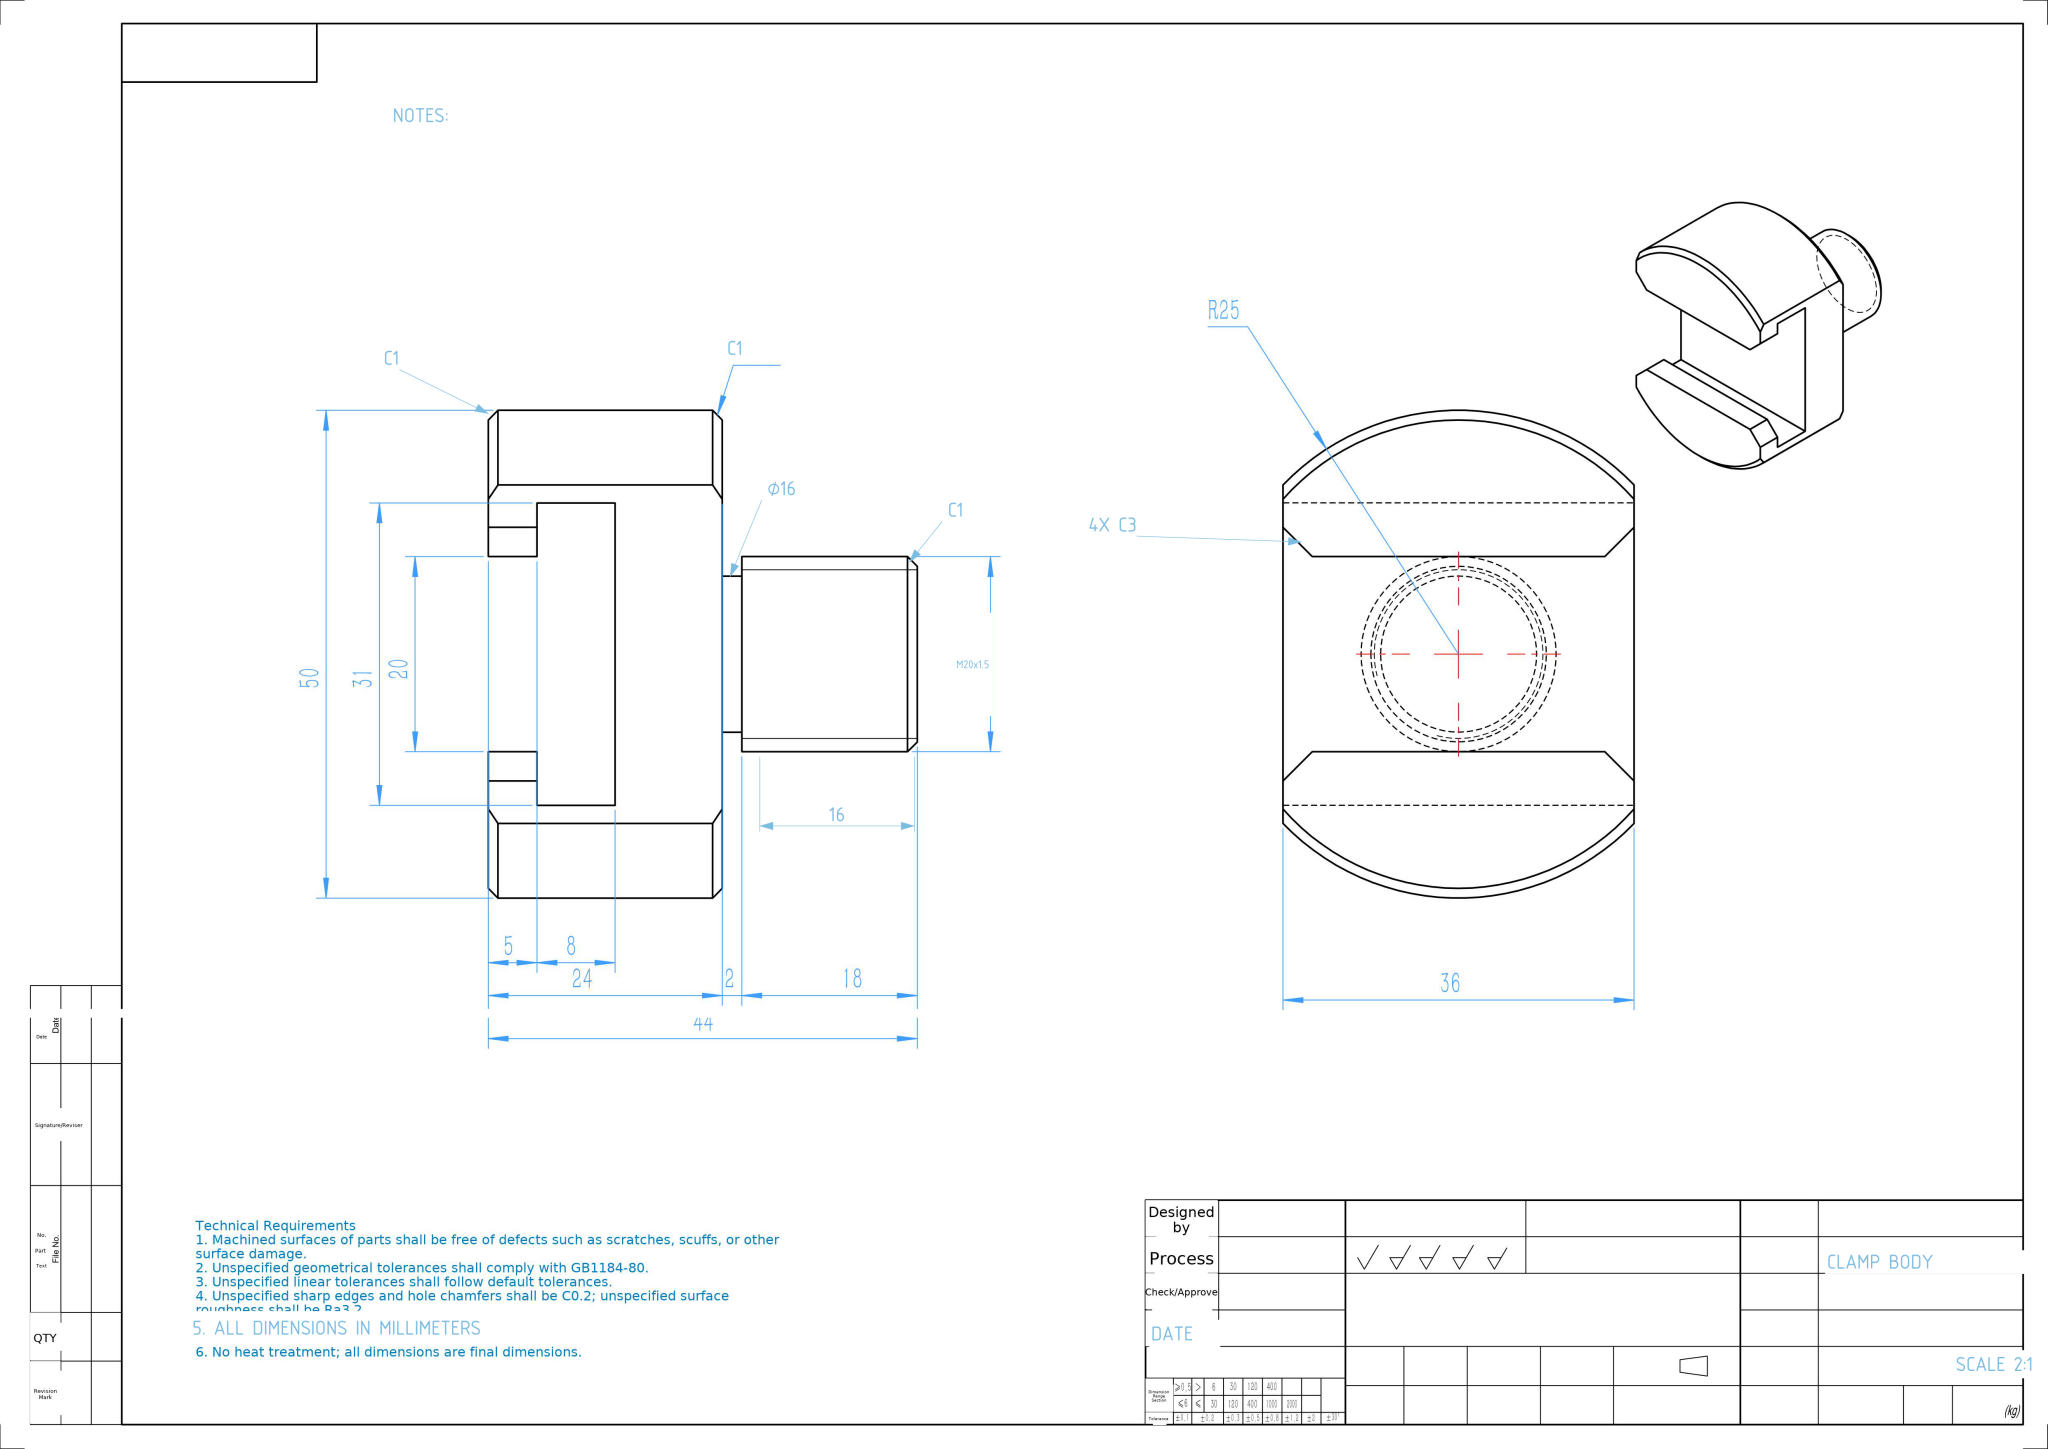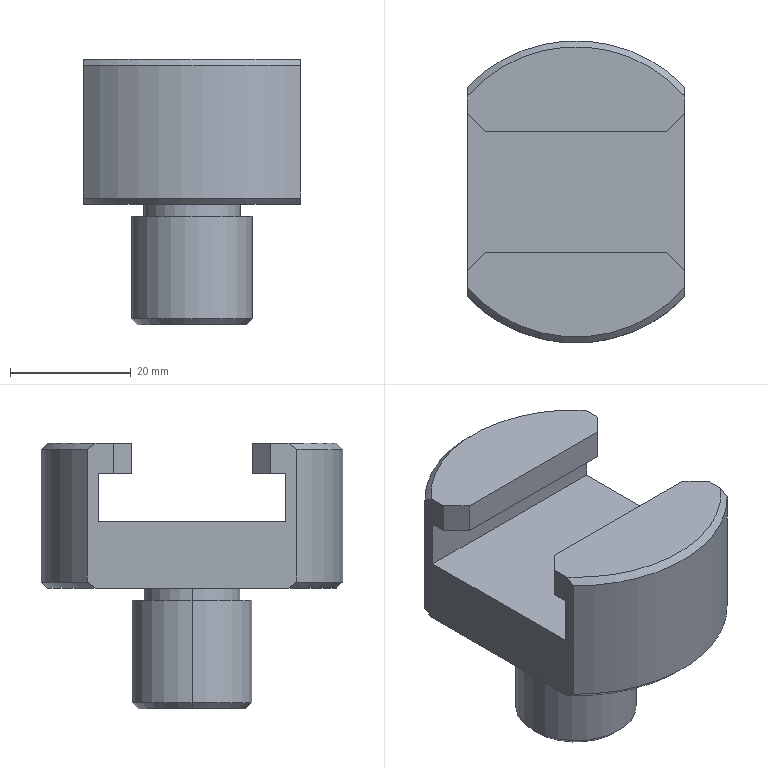Part | NX | mm | 1 solid | 30 faces | box 36 x 50 x 44 mm | volume 32432 mm3 | plane 18 | cylinder 6 | cone 6 | commonest cylinder face diameters 20 x2 16 x2 50 x2
STEP:
#1=CARTESIAN_POINT('',(10.,0.,-19.));
#2=VERTEX_POINT('',#1);
#3=CARTESIAN_POINT('',(-10.,0.,-19.));
#4=VERTEX_POINT('',#3);
#5=CARTESIAN_POINT('',(0.,0.,-19.));
#6=DIRECTION('',(0.,0.,1.));
#7=DIRECTION('',(-1.,0.,0.));
#8=AXIS2_PLACEMENT_3D('',#5,#6,#7);
#9=CIRCLE('',#8,10.);
#10=EDGE_CURVE('',#2,#4,#9,.T.);
#11=ORIENTED_EDGE('',*,*,#10,.T.);
#12=CARTESIAN_POINT('',(-10.,0.,-2.));
#13=VERTEX_POINT('',#12);
#14=CARTESIAN_POINT('',(-10.,0.,-20.));
#15=DIRECTION('',(0.,0.,1.));
#16=VECTOR('',#15,1000.);
#17=LINE('',#14,#16);
#18=EDGE_CURVE('',#4,#13,#17,.T.);
#19=ORIENTED_EDGE('',*,*,#18,.T.);
#20=CARTESIAN_POINT('',(10.,0.,-2.));
#21=VERTEX_POINT('',#20);
#22=CARTESIAN_POINT('',(0.,0.,-2.));
#23=DIRECTION('',(0.,0.,-1.));
#24=DIRECTION('',(-1.,0.,0.));
#25=AXIS2_PLACEMENT_3D('',#22,#23,#24);
#26=CIRCLE('',#25,10.);
#27=EDGE_CURVE('',#13,#21,#26,.T.);
#28=ORIENTED_EDGE('',*,*,#27,.T.);
#29=CARTESIAN_POINT('',(10.,0.,-20.));
#30=DIRECTION('',(0.,0.,1.));
#31=VECTOR('',#30,1000.);
#32=LINE('',#29,#31);
#33=EDGE_CURVE('',#2,#21,#32,.T.);
#34=ORIENTED_EDGE('',*,*,#33,.F.);
#35=EDGE_LOOP('',(#11,#19,#28,#34));
#36=FACE_OUTER_BOUND('',#35,.T.);
#37=CARTESIAN_POINT('',(0.,0.,-20.));
#38=DIRECTION('',(0.,0.,1.));
#39=DIRECTION('',(1.,0.,0.));
#40=AXIS2_PLACEMENT_3D('',#37,#38,#39);
#41=CYLINDRICAL_SURFACE('',#40,10.);
#42=ADVANCED_FACE('',(#36),#41,.T.);
#43=CARTESIAN_POINT('',(-9.,0.,-20.));
#44=VERTEX_POINT('',#43);
#45=CARTESIAN_POINT('',(9.,0.,-20.));
#46=VERTEX_POINT('',#45);
#47=CARTESIAN_POINT('',(0.,0.,-20.));
#48=DIRECTION('',(0.,0.,-1.));
#49=DIRECTION('',(-1.,0.,0.));
#50=AXIS2_PLACEMENT_3D('',#47,#48,#49);
#51=CIRCLE('',#50,9.);
#52=EDGE_CURVE('',#44,#46,#51,.T.);
#53=ORIENTED_EDGE('',*,*,#52,.F.);
#54=CARTESIAN_POINT('',(-9.,0.,-20.));
#55=DIRECTION('',(-0.7071,0.,0.7071));
#56=VECTOR('',#55,1000.);
#57=LINE('',#54,#56);
#58=EDGE_CURVE('',#44,#4,#57,.T.);
#59=ORIENTED_EDGE('',*,*,#58,.T.);
#60=ORIENTED_EDGE('',*,*,#10,.F.);
#61=CARTESIAN_POINT('',(9.,0.,-20.));
#62=DIRECTION('',(0.7071,0.,0.7071));
#63=VECTOR('',#62,1000.);
#64=LINE('',#61,#63);
#65=EDGE_CURVE('',#46,#2,#64,.T.);
#66=ORIENTED_EDGE('',*,*,#65,.F.);
#67=EDGE_LOOP('',(#53,#59,#60,#66));
#68=FACE_OUTER_BOUND('',#67,.T.);
#69=CARTESIAN_POINT('',(0.,0.,-20.));
#70=DIRECTION('',(0.,0.,1.));
#71=DIRECTION('',(1.,0.,0.));
#72=AXIS2_PLACEMENT_3D('',#69,#70,#71);
#73=CONICAL_SURFACE('',#72,9.,0.7854);
#74=ADVANCED_FACE('',(#68),#73,.T.);
#75=CARTESIAN_POINT('',(-8.,0.,0.));
#76=VERTEX_POINT('',#75);
#77=CARTESIAN_POINT('',(8.,0.,0.));
#78=VERTEX_POINT('',#77);
#79=CARTESIAN_POINT('',(0.,0.,0.));
#80=DIRECTION('',(0.,0.,-1.));
#81=DIRECTION('',(-1.,0.,0.));
#82=AXIS2_PLACEMENT_3D('',#79,#80,#81);
#83=CIRCLE('',#82,8.);
#84=EDGE_CURVE('',#76,#78,#83,.T.);
#85=ORIENTED_EDGE('',*,*,#84,.T.);
#86=CARTESIAN_POINT('',(8.,0.,-2.));
#87=VERTEX_POINT('',#86);
#88=CARTESIAN_POINT('',(8.,0.,-19.));
#89=DIRECTION('',(0.,0.,-1.));
#90=VECTOR('',#89,1000.);
#91=LINE('',#88,#90);
#92=EDGE_CURVE('',#78,#87,#91,.T.);
#93=ORIENTED_EDGE('',*,*,#92,.T.);
#94=CARTESIAN_POINT('',(-8.,0.,-2.));
#95=VERTEX_POINT('',#94);
#96=CARTESIAN_POINT('',(0.,0.,-2.));
#97=DIRECTION('',(0.,0.,-1.));
#98=DIRECTION('',(-1.,0.,0.));
#99=AXIS2_PLACEMENT_3D('',#96,#97,#98);
#100=CIRCLE('',#99,8.);
#101=EDGE_CURVE('',#95,#87,#100,.T.);
#102=ORIENTED_EDGE('',*,*,#101,.F.);
#103=CARTESIAN_POINT('',(-8.,0.,-19.));
#104=DIRECTION('',(0.,0.,-1.));
#105=VECTOR('',#104,1000.);
#106=LINE('',#103,#105);
#107=EDGE_CURVE('',#76,#95,#106,.T.);
#108=ORIENTED_EDGE('',*,*,#107,.F.);
#109=EDGE_LOOP('',(#85,#93,#102,#108));
#110=FACE_OUTER_BOUND('',#109,.T.);
#111=CARTESIAN_POINT('',(0.,0.,-19.));
#112=DIRECTION('',(0.,0.,-1.));
#113=DIRECTION('',(-1.,0.,0.));
#114=AXIS2_PLACEMENT_3D('',#111,#112,#113);
#115=CYLINDRICAL_SURFACE('',#114,8.);
#116=ADVANCED_FACE('',(#110),#115,.T.);
#117=CARTESIAN_POINT('',(18.,-17.349,1.));
#118=VERTEX_POINT('',#117);
#119=CARTESIAN_POINT('',(18.,-17.349,23.));
#120=VERTEX_POINT('',#119);
#121=CARTESIAN_POINT('',(18.,-17.349,24.));
#122=DIRECTION('',(0.,0.,1.));
#123=VECTOR('',#122,1000.);
#124=LINE('',#121,#123);
#125=EDGE_CURVE('',#118,#120,#124,.T.);
#126=ORIENTED_EDGE('',*,*,#125,.T.);
#127=CARTESIAN_POINT('',(-18.,-17.349,23.));
#128=VERTEX_POINT('',#127);
#129=CARTESIAN_POINT('',(0.,0.,23.));
#130=DIRECTION('',(0.,0.,-1.));
#131=DIRECTION('',(1.,0.,0.));
#132=AXIS2_PLACEMENT_3D('',#129,#130,#131);
#133=CIRCLE('',#132,25.);
#134=EDGE_CURVE('',#120,#128,#133,.T.);
#135=ORIENTED_EDGE('',*,*,#134,.T.);
#136=CARTESIAN_POINT('',(-18.,-17.349,1.));
#137=VERTEX_POINT('',#136);
#138=CARTESIAN_POINT('',(-18.,-17.349,24.));
#139=DIRECTION('',(0.,0.,-1.));
#140=VECTOR('',#139,1000.);
#141=LINE('',#138,#140);
#142=EDGE_CURVE('',#128,#137,#141,.T.);
#143=ORIENTED_EDGE('',*,*,#142,.T.);
#144=CARTESIAN_POINT('',(0.,0.,1.));
#145=DIRECTION('',(0.,0.,1.));
#146=DIRECTION('',(1.,0.,0.));
#147=AXIS2_PLACEMENT_3D('',#144,#145,#146);
#148=CIRCLE('',#147,25.);
#149=EDGE_CURVE('',#137,#118,#148,.T.);
#150=ORIENTED_EDGE('',*,*,#149,.T.);
#151=EDGE_LOOP('',(#126,#135,#143,#150));
#152=FACE_OUTER_BOUND('',#151,.T.);
#153=CARTESIAN_POINT('',(0.,0.,24.));
#154=DIRECTION('',(0.,0.,-1.));
#155=DIRECTION('',(-1.,0.,0.));
#156=AXIS2_PLACEMENT_3D('',#153,#154,#155);
#157=CYLINDRICAL_SURFACE('',#156,25.);
#158=ADVANCED_FACE('',(#152),#157,.T.);
#159=CARTESIAN_POINT('',(-18.,13.,24.));
#160=VERTEX_POINT('',#159);
#161=CARTESIAN_POINT('',(-18.,15.875,24.));
#162=VERTEX_POINT('',#161);
#163=CARTESIAN_POINT('',(-18.,25.313,24.));
#164=DIRECTION('',(0.,1.,0.));
#165=VECTOR('',#164,1000.);
#166=LINE('',#163,#165);
#167=EDGE_CURVE('',#160,#162,#166,.T.);
#168=ORIENTED_EDGE('',*,*,#167,.F.);
#169=CARTESIAN_POINT('',(-15.,10.,24.));
#170=VERTEX_POINT('',#169);
#171=CARTESIAN_POINT('',(-2.5,-2.5,24.));
#172=DIRECTION('',(0.7071,-0.7071,0.));
#173=VECTOR('',#172,1000.);
#174=LINE('',#171,#173);
#175=EDGE_CURVE('',#160,#170,#174,.T.);
#176=ORIENTED_EDGE('',*,*,#175,.T.);
#177=CARTESIAN_POINT('',(15.,10.,24.));
#178=VERTEX_POINT('',#177);
#179=CARTESIAN_POINT('',(0.,10.,24.));
#180=DIRECTION('',(-1.,0.,0.));
#181=VECTOR('',#180,1000.);
#182=LINE('',#179,#181);
#183=EDGE_CURVE('',#178,#170,#182,.T.);
#184=ORIENTED_EDGE('',*,*,#183,.F.);
#185=CARTESIAN_POINT('',(18.,13.,24.));
#186=VERTEX_POINT('',#185);
#187=CARTESIAN_POINT('',(2.5,-2.5,24.));
#188=DIRECTION('',(0.7071,0.7071,0.));
#189=VECTOR('',#188,1000.);
#190=LINE('',#187,#189);
#191=EDGE_CURVE('',#178,#186,#190,.T.);
#192=ORIENTED_EDGE('',*,*,#191,.T.);
#193=CARTESIAN_POINT('',(18.,15.875,24.));
#194=VERTEX_POINT('',#193);
#195=CARTESIAN_POINT('',(18.,25.314,24.));
#196=DIRECTION('',(0.,-1.,0.));
#197=VECTOR('',#196,1000.);
#198=LINE('',#195,#197);
#199=EDGE_CURVE('',#194,#186,#198,.T.);
#200=ORIENTED_EDGE('',*,*,#199,.F.);
#201=CARTESIAN_POINT('',(0.,0.,24.));
#202=DIRECTION('',(0.,0.,1.));
#203=DIRECTION('',(1.,0.,0.));
#204=AXIS2_PLACEMENT_3D('',#201,#202,#203);
#205=CIRCLE('',#204,24.);
#206=EDGE_CURVE('',#194,#162,#205,.T.);
#207=ORIENTED_EDGE('',*,*,#206,.T.);
#208=EDGE_LOOP('',(#168,#176,#184,#192,#200,#207));
#209=FACE_OUTER_BOUND('',#208,.T.);
#210=CARTESIAN_POINT('',(0.,0.,24.));
#211=DIRECTION('',(0.,0.,1.));
#212=DIRECTION('',(1.,0.,0.));
#213=AXIS2_PLACEMENT_3D('',#210,#211,#212);
#214=PLANE('',#213);
#215=ADVANCED_FACE('',(#209),#214,.T.);
#216=CARTESIAN_POINT('',(-18.,17.349,1.));
#217=VERTEX_POINT('',#216);
#218=CARTESIAN_POINT('',(-18.,17.349,23.));
#219=VERTEX_POINT('',#218);
#220=CARTESIAN_POINT('',(-18.,17.349,24.));
#221=DIRECTION('',(0.,0.,1.));
#222=VECTOR('',#221,1000.);
#223=LINE('',#220,#222);
#224=EDGE_CURVE('',#217,#219,#223,.T.);
#225=ORIENTED_EDGE('',*,*,#224,.T.);
#226=CARTESIAN_POINT('',(18.,17.349,23.));
#227=VERTEX_POINT('',#226);
#228=CARTESIAN_POINT('',(0.,0.,23.));
#229=DIRECTION('',(0.,0.,-1.));
#230=DIRECTION('',(1.,0.,0.));
#231=AXIS2_PLACEMENT_3D('',#228,#229,#230);
#232=CIRCLE('',#231,25.);
#233=EDGE_CURVE('',#219,#227,#232,.T.);
#234=ORIENTED_EDGE('',*,*,#233,.T.);
#235=CARTESIAN_POINT('',(18.,17.349,1.));
#236=VERTEX_POINT('',#235);
#237=CARTESIAN_POINT('',(18.,17.349,24.));
#238=DIRECTION('',(0.,0.,-1.));
#239=VECTOR('',#238,1000.);
#240=LINE('',#237,#239);
#241=EDGE_CURVE('',#227,#236,#240,.T.);
#242=ORIENTED_EDGE('',*,*,#241,.T.);
#243=CARTESIAN_POINT('',(0.,0.,1.));
#244=DIRECTION('',(0.,0.,1.));
#245=DIRECTION('',(1.,0.,0.));
#246=AXIS2_PLACEMENT_3D('',#243,#244,#245);
#247=CIRCLE('',#246,25.);
#248=EDGE_CURVE('',#236,#217,#247,.T.);
#249=ORIENTED_EDGE('',*,*,#248,.T.);
#250=EDGE_LOOP('',(#225,#234,#242,#249));
#251=FACE_OUTER_BOUND('',#250,.T.);
#252=CARTESIAN_POINT('',(0.,0.,24.));
#253=DIRECTION('',(0.,0.,-1.));
#254=DIRECTION('',(-1.,0.,0.));
#255=AXIS2_PLACEMENT_3D('',#252,#253,#254);
#256=CYLINDRICAL_SURFACE('',#255,25.);
#257=ADVANCED_FACE('',(#251),#256,.T.);
#258=CARTESIAN_POINT('',(-15.,-10.,24.));
#259=VERTEX_POINT('',#258);
#260=CARTESIAN_POINT('',(15.,-10.,24.));
#261=VERTEX_POINT('',#260);
#262=CARTESIAN_POINT('',(0.,-10.,24.));
#263=DIRECTION('',(1.,0.,0.));
#264=VECTOR('',#263,1000.);
#265=LINE('',#262,#264);
#266=EDGE_CURVE('',#259,#261,#265,.T.);
#267=ORIENTED_EDGE('',*,*,#266,.F.);
#268=CARTESIAN_POINT('',(-18.,-13.,24.));
#269=VERTEX_POINT('',#268);
#270=CARTESIAN_POINT('',(-2.5,2.5,24.));
#271=DIRECTION('',(-0.7071,-0.7071,0.));
#272=VECTOR('',#271,1000.);
#273=LINE('',#270,#272);
#274=EDGE_CURVE('',#259,#269,#273,.T.);
#275=ORIENTED_EDGE('',*,*,#274,.T.);
#276=CARTESIAN_POINT('',(-18.,-15.875,24.));
#277=VERTEX_POINT('',#276);
#278=CARTESIAN_POINT('',(-18.,25.313,24.));
#279=DIRECTION('',(0.,1.,0.));
#280=VECTOR('',#279,1000.);
#281=LINE('',#278,#280);
#282=EDGE_CURVE('',#277,#269,#281,.T.);
#283=ORIENTED_EDGE('',*,*,#282,.F.);
#284=CARTESIAN_POINT('',(18.,-15.875,24.));
#285=VERTEX_POINT('',#284);
#286=CARTESIAN_POINT('',(0.,0.,24.));
#287=DIRECTION('',(0.,0.,1.));
#288=DIRECTION('',(1.,0.,0.));
#289=AXIS2_PLACEMENT_3D('',#286,#287,#288);
#290=CIRCLE('',#289,24.);
#291=EDGE_CURVE('',#277,#285,#290,.T.);
#292=ORIENTED_EDGE('',*,*,#291,.T.);
#293=CARTESIAN_POINT('',(18.,-13.,24.));
#294=VERTEX_POINT('',#293);
#295=CARTESIAN_POINT('',(18.,25.314,24.));
#296=DIRECTION('',(0.,-1.,0.));
#297=VECTOR('',#296,1000.);
#298=LINE('',#295,#297);
#299=EDGE_CURVE('',#294,#285,#298,.T.);
#300=ORIENTED_EDGE('',*,*,#299,.F.);
#301=CARTESIAN_POINT('',(2.5,2.5,24.));
#302=DIRECTION('',(-0.7071,0.7071,0.));
#303=VECTOR('',#302,1000.);
#304=LINE('',#301,#303);
#305=EDGE_CURVE('',#294,#261,#304,.T.);
#306=ORIENTED_EDGE('',*,*,#305,.T.);
#307=EDGE_LOOP('',(#267,#275,#283,#292,#300,#306));
#308=FACE_OUTER_BOUND('',#307,.T.);
#309=CARTESIAN_POINT('',(0.,0.,24.));
#310=DIRECTION('',(0.,0.,1.));
#311=DIRECTION('',(1.,0.,0.));
#312=AXIS2_PLACEMENT_3D('',#309,#310,#311);
#313=PLANE('',#312);
#314=ADVANCED_FACE('',(#308),#313,.T.);
#315=CARTESIAN_POINT('',(18.,15.875,0.));
#316=VERTEX_POINT('',#315);
#317=CARTESIAN_POINT('',(18.,-15.875,0.));
#318=VERTEX_POINT('',#317);
#319=CARTESIAN_POINT('',(18.,0.,0.));
#320=DIRECTION('',(0.,-1.,0.));
#321=VECTOR('',#320,1000.);
#322=LINE('',#319,#321);
#323=EDGE_CURVE('',#316,#318,#322,.T.);
#324=ORIENTED_EDGE('',*,*,#323,.T.);
#325=CARTESIAN_POINT('',(-18.,-15.875,0.));
#326=VERTEX_POINT('',#325);
#327=CARTESIAN_POINT('',(0.,0.,0.));
#328=DIRECTION('',(0.,0.,-1.));
#329=DIRECTION('',(1.,0.,0.));
#330=AXIS2_PLACEMENT_3D('',#327,#328,#329);
#331=CIRCLE('',#330,24.);
#332=EDGE_CURVE('',#318,#326,#331,.T.);
#333=ORIENTED_EDGE('',*,*,#332,.T.);
#334=CARTESIAN_POINT('',(-18.,15.875,0.));
#335=VERTEX_POINT('',#334);
#336=CARTESIAN_POINT('',(-18.,0.,0.));
#337=DIRECTION('',(0.,1.,0.));
#338=VECTOR('',#337,1000.);
#339=LINE('',#336,#338);
#340=EDGE_CURVE('',#326,#335,#339,.T.);
#341=ORIENTED_EDGE('',*,*,#340,.T.);
#342=CARTESIAN_POINT('',(0.,0.,0.));
#343=DIRECTION('',(0.,0.,-1.));
#344=DIRECTION('',(1.,0.,0.));
#345=AXIS2_PLACEMENT_3D('',#342,#343,#344);
#346=CIRCLE('',#345,24.);
#347=EDGE_CURVE('',#335,#316,#346,.T.);
#348=ORIENTED_EDGE('',*,*,#347,.T.);
#349=EDGE_LOOP('',(#324,#333,#341,#348));
#350=FACE_OUTER_BOUND('',#349,.T.);
#351=ORIENTED_EDGE('',*,*,#84,.F.);
#352=CARTESIAN_POINT('',(0.,0.,0.));
#353=DIRECTION('',(0.,0.,-1.));
#354=DIRECTION('',(-1.,0.,0.));
#355=AXIS2_PLACEMENT_3D('',#352,#353,#354);
#356=CIRCLE('',#355,8.);
#357=EDGE_CURVE('',#78,#76,#356,.T.);
#358=ORIENTED_EDGE('',*,*,#357,.F.);
#359=EDGE_LOOP('',(#351,#358));
#360=FACE_BOUND('',#359,.T.);
#361=CARTESIAN_POINT('',(0.,0.,0.));
#362=DIRECTION('',(0.,0.,1.));
#363=DIRECTION('',(1.,0.,0.));
#364=AXIS2_PLACEMENT_3D('',#361,#362,#363);
#365=PLANE('',#364);
#366=ADVANCED_FACE('',(#350,#360),#365,.F.);
#367=CARTESIAN_POINT('',(-15.,10.,19.));
#368=VERTEX_POINT('',#367);
#369=CARTESIAN_POINT('',(15.,10.,19.));
#370=VERTEX_POINT('',#369);
#371=CARTESIAN_POINT('',(-50.,10.,19.));
#372=DIRECTION('',(1.,0.,0.));
#373=VECTOR('',#372,1000.);
#374=LINE('',#371,#373);
#375=EDGE_CURVE('',#368,#370,#374,.T.);
#376=ORIENTED_EDGE('',*,*,#375,.F.);
#377=CARTESIAN_POINT('',(-18.,13.,19.));
#378=VERTEX_POINT('',#377);
#379=CARTESIAN_POINT('',(-15.,10.,19.));
#380=DIRECTION('',(-0.7071,0.7071,0.));
#381=VECTOR('',#380,1000.);
#382=LINE('',#379,#381);
#383=EDGE_CURVE('',#368,#378,#382,.T.);
#384=ORIENTED_EDGE('',*,*,#383,.T.);
#385=CARTESIAN_POINT('',(-18.,15.5,19.));
#386=VERTEX_POINT('',#385);
#387=CARTESIAN_POINT('',(-18.,10.,19.));
#388=DIRECTION('',(0.,1.,0.));
#389=VECTOR('',#388,1000.);
#390=LINE('',#387,#389);
#391=EDGE_CURVE('',#378,#386,#390,.T.);
#392=ORIENTED_EDGE('',*,*,#391,.T.);
#393=CARTESIAN_POINT('',(18.,15.5,19.));
#394=VERTEX_POINT('',#393);
#395=CARTESIAN_POINT('',(-50.,15.5,19.));
#396=DIRECTION('',(1.,0.,0.));
#397=VECTOR('',#396,1000.);
#398=LINE('',#395,#397);
#399=EDGE_CURVE('',#386,#394,#398,.T.);
#400=ORIENTED_EDGE('',*,*,#399,.T.);
#401=CARTESIAN_POINT('',(18.,13.,19.));
#402=VERTEX_POINT('',#401);
#403=CARTESIAN_POINT('',(18.,10.,19.));
#404=DIRECTION('',(0.,-1.,-0.));
#405=VECTOR('',#404,1000.);
#406=LINE('',#403,#405);
#407=EDGE_CURVE('',#394,#402,#406,.T.);
#408=ORIENTED_EDGE('',*,*,#407,.T.);
#409=CARTESIAN_POINT('',(15.,10.,19.));
#410=DIRECTION('',(-0.7071,-0.7071,-0.));
#411=VECTOR('',#410,1000.);
#412=LINE('',#409,#411);
#413=EDGE_CURVE('',#402,#370,#412,.T.);
#414=ORIENTED_EDGE('',*,*,#413,.T.);
#415=EDGE_LOOP('',(#376,#384,#392,#400,#408,#414));
#416=FACE_OUTER_BOUND('',#415,.T.);
#417=CARTESIAN_POINT('',(-50.,10.,19.));
#418=DIRECTION('',(0.,-0.,1.));
#419=DIRECTION('',(0.,-1.,-0.));
#420=AXIS2_PLACEMENT_3D('',#417,#418,#419);
#421=PLANE('',#420);
#422=ADVANCED_FACE('',(#416),#421,.F.);
#423=ORIENTED_EDGE('',*,*,#399,.F.);
#424=CARTESIAN_POINT('',(-18.,15.5,11.));
#425=VERTEX_POINT('',#424);
#426=CARTESIAN_POINT('',(-18.,15.5,19.));
#427=DIRECTION('',(0.,-0.,-1.));
#428=VECTOR('',#427,1000.);
#429=LINE('',#426,#428);
#430=EDGE_CURVE('',#386,#425,#429,.T.);
#431=ORIENTED_EDGE('',*,*,#430,.T.);
#432=CARTESIAN_POINT('',(18.,15.5,11.));
#433=VERTEX_POINT('',#432);
#434=CARTESIAN_POINT('',(-50.,15.5,11.));
#435=DIRECTION('',(1.,0.,0.));
#436=VECTOR('',#435,1000.);
#437=LINE('',#434,#436);
#438=EDGE_CURVE('',#425,#433,#437,.T.);
#439=ORIENTED_EDGE('',*,*,#438,.T.);
#440=CARTESIAN_POINT('',(18.,15.5,19.));
#441=DIRECTION('',(0.,0.,1.));
#442=VECTOR('',#441,1000.);
#443=LINE('',#440,#442);
#444=EDGE_CURVE('',#433,#394,#443,.T.);
#445=ORIENTED_EDGE('',*,*,#444,.T.);
#446=EDGE_LOOP('',(#423,#431,#439,#445));
#447=FACE_OUTER_BOUND('',#446,.T.);
#448=CARTESIAN_POINT('',(-50.,15.5,19.));
#449=DIRECTION('',(0.,1.,-0.));
#450=DIRECTION('',(0.,0.,1.));
#451=AXIS2_PLACEMENT_3D('',#448,#449,#450);
#452=PLANE('',#451);
#453=ADVANCED_FACE('',(#447),#452,.F.);
#454=ORIENTED_EDGE('',*,*,#438,.F.);
#455=CARTESIAN_POINT('',(-18.,-15.5,11.));
#456=VERTEX_POINT('',#455);
#457=CARTESIAN_POINT('',(-18.,15.5,11.));
#458=DIRECTION('',(0.,-1.,0.));
#459=VECTOR('',#458,1000.);
#460=LINE('',#457,#459);
#461=EDGE_CURVE('',#425,#456,#460,.T.);
#462=ORIENTED_EDGE('',*,*,#461,.T.);
#463=CARTESIAN_POINT('',(18.,-15.5,11.));
#464=VERTEX_POINT('',#463);
#465=CARTESIAN_POINT('',(-50.,-15.5,11.));
#466=DIRECTION('',(1.,0.,0.));
#467=VECTOR('',#466,1000.);
#468=LINE('',#465,#467);
#469=EDGE_CURVE('',#456,#464,#468,.T.);
#470=ORIENTED_EDGE('',*,*,#469,.T.);
#471=CARTESIAN_POINT('',(18.,15.5,11.));
#472=DIRECTION('',(0.,1.,0.));
#473=VECTOR('',#472,1000.);
#474=LINE('',#471,#473);
#475=EDGE_CURVE('',#464,#433,#474,.T.);
#476=ORIENTED_EDGE('',*,*,#475,.T.);
#477=EDGE_LOOP('',(#454,#462,#470,#476));
#478=FACE_OUTER_BOUND('',#477,.T.);
#479=CARTESIAN_POINT('',(-50.,15.5,11.));
#480=DIRECTION('',(0.,0.,-1.));
#481=DIRECTION('',(-1.,0.,0.));
#482=AXIS2_PLACEMENT_3D('',#479,#480,#481);
#483=PLANE('',#482);
#484=ADVANCED_FACE('',(#478),#483,.F.);
#485=ORIENTED_EDGE('',*,*,#469,.F.);
#486=CARTESIAN_POINT('',(-18.,-15.5,19.));
#487=VERTEX_POINT('',#486);
#488=CARTESIAN_POINT('',(-18.,-15.5,11.));
#489=DIRECTION('',(0.,-0.,1.));
#490=VECTOR('',#489,1000.);
#491=LINE('',#488,#490);
#492=EDGE_CURVE('',#456,#487,#491,.T.);
#493=ORIENTED_EDGE('',*,*,#492,.T.);
#494=CARTESIAN_POINT('',(18.,-15.5,19.));
#495=VERTEX_POINT('',#494);
#496=CARTESIAN_POINT('',(-50.,-15.5,19.));
#497=DIRECTION('',(1.,0.,0.));
#498=VECTOR('',#497,1000.);
#499=LINE('',#496,#498);
#500=EDGE_CURVE('',#487,#495,#499,.T.);
#501=ORIENTED_EDGE('',*,*,#500,.T.);
#502=CARTESIAN_POINT('',(18.,-15.5,11.));
#503=DIRECTION('',(0.,0.,-1.));
#504=VECTOR('',#503,1000.);
#505=LINE('',#502,#504);
#506=EDGE_CURVE('',#495,#464,#505,.T.);
#507=ORIENTED_EDGE('',*,*,#506,.T.);
#508=EDGE_LOOP('',(#485,#493,#501,#507));
#509=FACE_OUTER_BOUND('',#508,.T.);
#510=CARTESIAN_POINT('',(-50.,-15.5,11.));
#511=DIRECTION('',(0.,-1.,-0.));
#512=DIRECTION('',(0.,0.,-1.));
#513=AXIS2_PLACEMENT_3D('',#510,#511,#512);
#514=PLANE('',#513);
#515=ADVANCED_FACE('',(#509),#514,.F.);
#516=CARTESIAN_POINT('',(-18.,-13.,19.));
#517=VERTEX_POINT('',#516);
#518=CARTESIAN_POINT('',(-18.,-15.5,19.));
#519=DIRECTION('',(0.,1.,-0.));
#520=VECTOR('',#519,1000.);
#521=LINE('',#518,#520);
#522=EDGE_CURVE('',#487,#517,#521,.T.);
#523=ORIENTED_EDGE('',*,*,#522,.T.);
#524=CARTESIAN_POINT('',(-15.,-10.,19.));
#525=VERTEX_POINT('',#524);
#526=CARTESIAN_POINT('',(-15.,-10.,19.));
#527=DIRECTION('',(0.7071,0.7071,-0.));
#528=VECTOR('',#527,1000.);
#529=LINE('',#526,#528);
#530=EDGE_CURVE('',#517,#525,#529,.T.);
#531=ORIENTED_EDGE('',*,*,#530,.T.);
#532=CARTESIAN_POINT('',(15.,-10.,19.));
#533=VERTEX_POINT('',#532);
#534=CARTESIAN_POINT('',(-50.,-10.,19.));
#535=DIRECTION('',(1.,0.,0.));
#536=VECTOR('',#535,1000.);
#537=LINE('',#534,#536);
#538=EDGE_CURVE('',#525,#533,#537,.T.);
#539=ORIENTED_EDGE('',*,*,#538,.T.);
#540=CARTESIAN_POINT('',(18.,-13.,19.));
#541=VERTEX_POINT('',#540);
#542=CARTESIAN_POINT('',(15.,-10.,19.));
#543=DIRECTION('',(0.7071,-0.7071,0.));
#544=VECTOR('',#543,1000.);
#545=LINE('',#542,#544);
#546=EDGE_CURVE('',#533,#541,#545,.T.);
#547=ORIENTED_EDGE('',*,*,#546,.T.);
#548=CARTESIAN_POINT('',(18.,-15.5,19.));
#549=DIRECTION('',(0.,-1.,0.));
#550=VECTOR('',#549,1000.);
#551=LINE('',#548,#550);
#552=EDGE_CURVE('',#541,#495,#551,.T.);
#553=ORIENTED_EDGE('',*,*,#552,.T.);
#554=ORIENTED_EDGE('',*,*,#500,.F.);
#555=EDGE_LOOP('',(#523,#531,#539,#547,#553,#554));
#556=FACE_OUTER_BOUND('',#555,.T.);
#557=CARTESIAN_POINT('',(-50.,-15.5,19.));
#558=DIRECTION('',(0.,0.,1.));
#559=DIRECTION('',(0.,-1.,0.));
#560=AXIS2_PLACEMENT_3D('',#557,#558,#559);
#561=PLANE('',#560);
#562=ADVANCED_FACE('',(#556),#561,.F.);
#563=ORIENTED_EDGE('',*,*,#183,.T.);
#564=CARTESIAN_POINT('',(-15.,10.,24.));
#565=DIRECTION('',(0.,0.,-1.));
#566=VECTOR('',#565,1000.);
#567=LINE('',#564,#566);
#568=EDGE_CURVE('',#170,#368,#567,.T.);
#569=ORIENTED_EDGE('',*,*,#568,.T.);
#570=ORIENTED_EDGE('',*,*,#375,.T.);
#571=CARTESIAN_POINT('',(15.,10.,24.));
#572=DIRECTION('',(0.,0.,1.));
#573=VECTOR('',#572,1000.);
#574=LINE('',#571,#573);
#575=EDGE_CURVE('',#370,#178,#574,.T.);
#576=ORIENTED_EDGE('',*,*,#575,.T.);
#577=EDGE_LOOP('',(#563,#569,#570,#576));
#578=FACE_OUTER_BOUND('',#577,.T.);
#579=CARTESIAN_POINT('',(-50.,10.,24.));
#580=DIRECTION('',(0.,1.,0.));
#581=DIRECTION('',(0.,0.,1.));
#582=AXIS2_PLACEMENT_3D('',#579,#580,#581);
#583=PLANE('',#582);
#584=ADVANCED_FACE('',(#578),#583,.F.);
#585=ORIENTED_EDGE('',*,*,#538,.F.);
#586=CARTESIAN_POINT('',(-15.,-10.,19.));
#587=DIRECTION('',(0.,0.,1.));
#588=VECTOR('',#587,1000.);
#589=LINE('',#586,#588);
#590=EDGE_CURVE('',#525,#259,#589,.T.);
#591=ORIENTED_EDGE('',*,*,#590,.T.);
#592=ORIENTED_EDGE('',*,*,#266,.T.);
#593=CARTESIAN_POINT('',(15.,-10.,19.));
#594=DIRECTION('',(0.,0.,-1.));
#595=VECTOR('',#594,1000.);
#596=LINE('',#593,#595);
#597=EDGE_CURVE('',#261,#533,#596,.T.);
#598=ORIENTED_EDGE('',*,*,#597,.T.);
#599=EDGE_LOOP('',(#585,#591,#592,#598));
#600=FACE_OUTER_BOUND('',#599,.T.);
#601=CARTESIAN_POINT('',(-50.,-10.,19.));
#602=DIRECTION('',(0.,-1.,0.));
#603=DIRECTION('',(0.,0.,-1.));
#604=AXIS2_PLACEMENT_3D('',#601,#602,#603);
#605=PLANE('',#604);
#606=ADVANCED_FACE('',(#600),#605,.F.);
#607=ORIENTED_EDGE('',*,*,#199,.T.);
#608=CARTESIAN_POINT('',(18.,13.,-76.));
#609=DIRECTION('',(0.,0.,-1.));
#610=VECTOR('',#609,1000.);
#611=LINE('',#608,#610);
#612=EDGE_CURVE('',#186,#402,#611,.T.);
#613=ORIENTED_EDGE('',*,*,#612,.T.);
#614=ORIENTED_EDGE('',*,*,#407,.F.);
#615=ORIENTED_EDGE('',*,*,#444,.F.);
#616=ORIENTED_EDGE('',*,*,#475,.F.);
#617=ORIENTED_EDGE('',*,*,#506,.F.);
#618=ORIENTED_EDGE('',*,*,#552,.F.);
#619=CARTESIAN_POINT('',(18.,-13.,-76.));
#620=DIRECTION('',(0.,0.,1.));
#621=VECTOR('',#620,1000.);
#622=LINE('',#619,#621);
#623=EDGE_CURVE('',#541,#294,#622,.T.);
#624=ORIENTED_EDGE('',*,*,#623,.T.);
#625=ORIENTED_EDGE('',*,*,#299,.T.);
#626=CARTESIAN_POINT('',(18.,-15.875,24.));
#627=CARTESIAN_POINT('',(18.,-16.37,23.672));
#628=CARTESIAN_POINT('',(18.,-16.861,23.339));
#629=CARTESIAN_POINT('',(18.,-17.349,23.));
#630=B_SPLINE_CURVE_WITH_KNOTS('',3,(#626,#627,#628,#629),.UNSPECIFIED.,.F.,.F.,(4,4),(0.,0.001782),.UNSPECIFIED.);
#631=EDGE_CURVE('',#285,#120,#630,.T.);
#632=ORIENTED_EDGE('',*,*,#631,.T.);
#633=ORIENTED_EDGE('',*,*,#125,.F.);
#634=CARTESIAN_POINT('',(18.,-17.349,1.));
#635=CARTESIAN_POINT('',(18.,-16.861,0.6613));
#636=CARTESIAN_POINT('',(18.,-16.37,0.3277));
#637=CARTESIAN_POINT('',(18.,-15.875,0.));
#638=B_SPLINE_CURVE_WITH_KNOTS('',3,(#634,#635,#636,#637),.UNSPECIFIED.,.F.,.F.,(4,4),(0.,0.001782),.UNSPECIFIED.);
#639=EDGE_CURVE('',#118,#318,#638,.T.);
#640=ORIENTED_EDGE('',*,*,#639,.T.);
#641=ORIENTED_EDGE('',*,*,#323,.F.);
#642=CARTESIAN_POINT('',(18.,15.875,0.));
#643=CARTESIAN_POINT('',(18.,16.37,0.3277));
#644=CARTESIAN_POINT('',(18.,16.861,0.6613));
#645=CARTESIAN_POINT('',(18.,17.349,1.));
#646=B_SPLINE_CURVE_WITH_KNOTS('',3,(#642,#643,#644,#645),.UNSPECIFIED.,.F.,.F.,(4,4),(0.,0.001782),.UNSPECIFIED.);
#647=EDGE_CURVE('',#316,#236,#646,.T.);
#648=ORIENTED_EDGE('',*,*,#647,.T.);
#649=ORIENTED_EDGE('',*,*,#241,.F.);
#650=CARTESIAN_POINT('',(18.,17.349,23.));
#651=CARTESIAN_POINT('',(18.,16.861,23.339));
#652=CARTESIAN_POINT('',(18.,16.37,23.672));
#653=CARTESIAN_POINT('',(18.,15.875,24.));
#654=B_SPLINE_CURVE_WITH_KNOTS('',3,(#650,#651,#652,#653),.UNSPECIFIED.,.F.,.F.,(4,4),(0.,0.001782),.UNSPECIFIED.);
#655=EDGE_CURVE('',#227,#194,#654,.T.);
#656=ORIENTED_EDGE('',*,*,#655,.T.);
#657=EDGE_LOOP('',(#607,#613,#614,#615,#616,#617,#618,#624,#625,#632,#633,#640,#641,#648,#649,#656));
#658=FACE_OUTER_BOUND('',#657,.T.);
#659=CARTESIAN_POINT('',(18.,25.314,-76.));
#660=DIRECTION('',(-1.,0.,0.));
#661=DIRECTION('',(0.,0.,1.));
#662=AXIS2_PLACEMENT_3D('',#659,#660,#661);
#663=PLANE('',#662);
#664=ADVANCED_FACE('',(#658),#663,.F.);
#665=ORIENTED_EDGE('',*,*,#282,.T.);
#666=CARTESIAN_POINT('',(-18.,-13.,-76.));
#667=DIRECTION('',(0.,0.,-1.));
#668=VECTOR('',#667,1000.);
#669=LINE('',#666,#668);
#670=EDGE_CURVE('',#269,#517,#669,.T.);
#671=ORIENTED_EDGE('',*,*,#670,.T.);
#672=ORIENTED_EDGE('',*,*,#522,.F.);
#673=ORIENTED_EDGE('',*,*,#492,.F.);
#674=ORIENTED_EDGE('',*,*,#461,.F.);
#675=ORIENTED_EDGE('',*,*,#430,.F.);
#676=ORIENTED_EDGE('',*,*,#391,.F.);
#677=CARTESIAN_POINT('',(-18.,13.,-76.));
#678=DIRECTION('',(0.,0.,1.));
#679=VECTOR('',#678,1000.);
#680=LINE('',#677,#679);
#681=EDGE_CURVE('',#378,#160,#680,.T.);
#682=ORIENTED_EDGE('',*,*,#681,.T.);
#683=ORIENTED_EDGE('',*,*,#167,.T.);
#684=CARTESIAN_POINT('',(-18.,15.875,24.));
#685=CARTESIAN_POINT('',(-18.,16.37,23.672));
#686=CARTESIAN_POINT('',(-18.,16.861,23.339));
#687=CARTESIAN_POINT('',(-18.,17.349,23.));
#688=B_SPLINE_CURVE_WITH_KNOTS('',3,(#684,#685,#686,#687),.UNSPECIFIED.,.F.,.F.,(4,4),(0.,0.001782),.UNSPECIFIED.);
#689=EDGE_CURVE('',#162,#219,#688,.T.);
#690=ORIENTED_EDGE('',*,*,#689,.T.);
#691=ORIENTED_EDGE('',*,*,#224,.F.);
#692=CARTESIAN_POINT('',(-18.,17.349,1.));
#693=CARTESIAN_POINT('',(-18.,16.861,0.6613));
#694=CARTESIAN_POINT('',(-18.,16.37,0.3277));
#695=CARTESIAN_POINT('',(-18.,15.875,0.));
#696=B_SPLINE_CURVE_WITH_KNOTS('',3,(#692,#693,#694,#695),.UNSPECIFIED.,.F.,.F.,(4,4),(0.,0.001782),.UNSPECIFIED.);
#697=EDGE_CURVE('',#217,#335,#696,.T.);
#698=ORIENTED_EDGE('',*,*,#697,.T.);
#699=ORIENTED_EDGE('',*,*,#340,.F.);
#700=CARTESIAN_POINT('',(-18.,-15.875,0.));
#701=CARTESIAN_POINT('',(-18.,-16.37,0.3277));
#702=CARTESIAN_POINT('',(-18.,-16.861,0.6613));
#703=CARTESIAN_POINT('',(-18.,-17.349,1.));
#704=B_SPLINE_CURVE_WITH_KNOTS('',3,(#700,#701,#702,#703),.UNSPECIFIED.,.F.,.F.,(4,4),(0.,0.001782),.UNSPECIFIED.);
#705=EDGE_CURVE('',#326,#137,#704,.T.);
#706=ORIENTED_EDGE('',*,*,#705,.T.);
#707=ORIENTED_EDGE('',*,*,#142,.F.);
#708=CARTESIAN_POINT('',(-18.,-17.349,23.));
#709=CARTESIAN_POINT('',(-18.,-16.861,23.339));
#710=CARTESIAN_POINT('',(-18.,-16.37,23.672));
#711=CARTESIAN_POINT('',(-18.,-15.875,24.));
#712=B_SPLINE_CURVE_WITH_KNOTS('',3,(#708,#709,#710,#711),.UNSPECIFIED.,.F.,.F.,(4,4),(0.,0.001782),.UNSPECIFIED.);
#713=EDGE_CURVE('',#128,#277,#712,.T.);
#714=ORIENTED_EDGE('',*,*,#713,.T.);
#715=EDGE_LOOP('',(#665,#671,#672,#673,#674,#675,#676,#682,#683,#690,#691,#698,#699,#706,#707,#714));
#716=FACE_OUTER_BOUND('',#715,.T.);
#717=CARTESIAN_POINT('',(-18.,25.313,-76.));
#718=DIRECTION('',(1.,0.,0.));
#719=DIRECTION('',(0.,0.,-1.));
#720=AXIS2_PLACEMENT_3D('',#717,#718,#719);
#721=PLANE('',#720);
#722=ADVANCED_FACE('',(#716),#721,.F.);
#723=ORIENTED_EDGE('',*,*,#655,.F.);
#724=ORIENTED_EDGE('',*,*,#233,.F.);
#725=ORIENTED_EDGE('',*,*,#689,.F.);
#726=ORIENTED_EDGE('',*,*,#206,.F.);
#727=EDGE_LOOP('',(#723,#724,#725,#726));
#728=FACE_OUTER_BOUND('',#727,.T.);
#729=CARTESIAN_POINT('',(0.,0.,24.));
#730=DIRECTION('',(0.,0.,-1.));
#731=DIRECTION('',(-1.,0.,0.));
#732=AXIS2_PLACEMENT_3D('',#729,#730,#731);
#733=CONICAL_SURFACE('',#732,24.,0.7854);
#734=ADVANCED_FACE('',(#728),#733,.T.);
#735=ORIENTED_EDGE('',*,*,#713,.F.);
#736=ORIENTED_EDGE('',*,*,#134,.F.);
#737=ORIENTED_EDGE('',*,*,#631,.F.);
#738=ORIENTED_EDGE('',*,*,#291,.F.);
#739=EDGE_LOOP('',(#735,#736,#737,#738));
#740=FACE_OUTER_BOUND('',#739,.T.);
#741=CARTESIAN_POINT('',(0.,0.,24.));
#742=DIRECTION('',(0.,0.,-1.));
#743=DIRECTION('',(-1.,0.,0.));
#744=AXIS2_PLACEMENT_3D('',#741,#742,#743);
#745=CONICAL_SURFACE('',#744,24.,0.7854);
#746=ADVANCED_FACE('',(#740),#745,.T.);
#747=ORIENTED_EDGE('',*,*,#705,.F.);
#748=ORIENTED_EDGE('',*,*,#332,.F.);
#749=ORIENTED_EDGE('',*,*,#639,.F.);
#750=ORIENTED_EDGE('',*,*,#149,.F.);
#751=EDGE_LOOP('',(#747,#748,#749,#750));
#752=FACE_OUTER_BOUND('',#751,.T.);
#753=CARTESIAN_POINT('',(0.,0.,1.));
#754=DIRECTION('',(0.,0.,1.));
#755=DIRECTION('',(1.,0.,0.));
#756=AXIS2_PLACEMENT_3D('',#753,#754,#755);
#757=CONICAL_SURFACE('',#756,25.,0.7854);
#758=ADVANCED_FACE('',(#752),#757,.T.);
#759=ORIENTED_EDGE('',*,*,#647,.F.);
#760=ORIENTED_EDGE('',*,*,#347,.F.);
#761=ORIENTED_EDGE('',*,*,#697,.F.);
#762=ORIENTED_EDGE('',*,*,#248,.F.);
#763=EDGE_LOOP('',(#759,#760,#761,#762));
#764=FACE_OUTER_BOUND('',#763,.T.);
#765=CARTESIAN_POINT('',(0.,0.,1.));
#766=DIRECTION('',(0.,0.,1.));
#767=DIRECTION('',(1.,0.,0.));
#768=AXIS2_PLACEMENT_3D('',#765,#766,#767);
#769=CONICAL_SURFACE('',#768,25.,0.7854);
#770=ADVANCED_FACE('',(#764),#769,.T.);
#771=ORIENTED_EDGE('',*,*,#530,.F.);
#772=ORIENTED_EDGE('',*,*,#670,.F.);
#773=ORIENTED_EDGE('',*,*,#274,.F.);
#774=ORIENTED_EDGE('',*,*,#590,.F.);
#775=EDGE_LOOP('',(#771,#772,#773,#774));
#776=FACE_OUTER_BOUND('',#775,.T.);
#777=CARTESIAN_POINT('',(-15.,-10.,19.));
#778=DIRECTION('',(0.7071,-0.7071,0.));
#779=DIRECTION('',(0.,0.,1.));
#780=AXIS2_PLACEMENT_3D('',#777,#778,#779);
#781=PLANE('',#780);
#782=ADVANCED_FACE('',(#776),#781,.F.);
#783=ORIENTED_EDGE('',*,*,#175,.F.);
#784=ORIENTED_EDGE('',*,*,#681,.F.);
#785=ORIENTED_EDGE('',*,*,#383,.F.);
#786=ORIENTED_EDGE('',*,*,#568,.F.);
#787=EDGE_LOOP('',(#783,#784,#785,#786));
#788=FACE_OUTER_BOUND('',#787,.T.);
#789=CARTESIAN_POINT('',(-15.,10.,24.));
#790=DIRECTION('',(0.7071,0.7071,0.));
#791=DIRECTION('',(0.,0.,-1.));
#792=AXIS2_PLACEMENT_3D('',#789,#790,#791);
#793=PLANE('',#792);
#794=ADVANCED_FACE('',(#788),#793,.F.);
#795=ORIENTED_EDGE('',*,*,#413,.F.);
#796=ORIENTED_EDGE('',*,*,#612,.F.);
#797=ORIENTED_EDGE('',*,*,#191,.F.);
#798=ORIENTED_EDGE('',*,*,#575,.F.);
#799=EDGE_LOOP('',(#795,#796,#797,#798));
#800=FACE_OUTER_BOUND('',#799,.T.);
#801=CARTESIAN_POINT('',(15.,10.,24.));
#802=DIRECTION('',(-0.7071,0.7071,0.));
#803=DIRECTION('',(0.,0.,1.));
#804=AXIS2_PLACEMENT_3D('',#801,#802,#803);
#805=PLANE('',#804);
#806=ADVANCED_FACE('',(#800),#805,.F.);
#807=ORIENTED_EDGE('',*,*,#305,.F.);
#808=ORIENTED_EDGE('',*,*,#623,.F.);
#809=ORIENTED_EDGE('',*,*,#546,.F.);
#810=ORIENTED_EDGE('',*,*,#597,.F.);
#811=EDGE_LOOP('',(#807,#808,#809,#810));
#812=FACE_OUTER_BOUND('',#811,.T.);
#813=CARTESIAN_POINT('',(15.,-10.,19.));
#814=DIRECTION('',(-0.7071,-0.7071,0.));
#815=DIRECTION('',(0.,0.,-1.));
#816=AXIS2_PLACEMENT_3D('',#813,#814,#815);
#817=PLANE('',#816);
#818=ADVANCED_FACE('',(#812),#817,.F.);
#819=ORIENTED_EDGE('',*,*,#92,.F.);
#820=ORIENTED_EDGE('',*,*,#357,.T.);
#821=ORIENTED_EDGE('',*,*,#107,.T.);
#822=CARTESIAN_POINT('',(0.,0.,-2.));
#823=DIRECTION('',(0.,0.,-1.));
#824=DIRECTION('',(-1.,0.,0.));
#825=AXIS2_PLACEMENT_3D('',#822,#823,#824);
#826=CIRCLE('',#825,8.);
#827=EDGE_CURVE('',#87,#95,#826,.T.);
#828=ORIENTED_EDGE('',*,*,#827,.F.);
#829=EDGE_LOOP('',(#819,#820,#821,#828));
#830=FACE_OUTER_BOUND('',#829,.T.);
#831=CARTESIAN_POINT('',(0.,0.,-19.));
#832=DIRECTION('',(0.,0.,-1.));
#833=DIRECTION('',(-1.,0.,0.));
#834=AXIS2_PLACEMENT_3D('',#831,#832,#833);
#835=CYLINDRICAL_SURFACE('',#834,8.);
#836=ADVANCED_FACE('',(#830),#835,.T.);
#837=CARTESIAN_POINT('',(0.,0.,-2.));
#838=DIRECTION('',(0.,0.,-1.));
#839=DIRECTION('',(-1.,0.,0.));
#840=AXIS2_PLACEMENT_3D('',#837,#838,#839);
#841=CIRCLE('',#840,10.);
#842=EDGE_CURVE('',#21,#13,#841,.T.);
#843=ORIENTED_EDGE('',*,*,#842,.F.);
#844=ORIENTED_EDGE('',*,*,#27,.F.);
#845=EDGE_LOOP('',(#843,#844));
#846=FACE_OUTER_BOUND('',#845,.T.);
#847=ORIENTED_EDGE('',*,*,#101,.T.);
#848=ORIENTED_EDGE('',*,*,#827,.T.);
#849=EDGE_LOOP('',(#847,#848));
#850=FACE_BOUND('',#849,.T.);
#851=CARTESIAN_POINT('',(-8.,0.,-2.));
#852=DIRECTION('',(0.,0.,-1.));
#853=DIRECTION('',(-1.,0.,0.));
#854=AXIS2_PLACEMENT_3D('',#851,#852,#853);
#855=PLANE('',#854);
#856=ADVANCED_FACE('',(#846,#850),#855,.F.);
#857=CARTESIAN_POINT('',(0.,0.,-20.));
#858=DIRECTION('',(0.,0.,-1.));
#859=DIRECTION('',(-1.,0.,0.));
#860=AXIS2_PLACEMENT_3D('',#857,#858,#859);
#861=CIRCLE('',#860,9.);
#862=EDGE_CURVE('',#46,#44,#861,.T.);
#863=ORIENTED_EDGE('',*,*,#862,.T.);
#864=ORIENTED_EDGE('',*,*,#52,.T.);
#865=EDGE_LOOP('',(#863,#864));
#866=FACE_OUTER_BOUND('',#865,.T.);
#867=CARTESIAN_POINT('',(0.,0.,-20.));
#868=DIRECTION('',(0.,0.,-1.));
#869=DIRECTION('',(-1.,0.,0.));
#870=AXIS2_PLACEMENT_3D('',#867,#868,#869);
#871=PLANE('',#870);
#872=ADVANCED_FACE('',(#866),#871,.T.);
#873=ORIENTED_EDGE('',*,*,#58,.F.);
#874=ORIENTED_EDGE('',*,*,#862,.F.);
#875=ORIENTED_EDGE('',*,*,#65,.T.);
#876=CARTESIAN_POINT('',(0.,0.,-19.));
#877=DIRECTION('',(0.,0.,1.));
#878=DIRECTION('',(-1.,0.,0.));
#879=AXIS2_PLACEMENT_3D('',#876,#877,#878);
#880=CIRCLE('',#879,10.);
#881=EDGE_CURVE('',#4,#2,#880,.T.);
#882=ORIENTED_EDGE('',*,*,#881,.F.);
#883=EDGE_LOOP('',(#873,#874,#875,#882));
#884=FACE_OUTER_BOUND('',#883,.T.);
#885=CARTESIAN_POINT('',(0.,0.,-20.));
#886=DIRECTION('',(0.,0.,1.));
#887=DIRECTION('',(1.,0.,0.));
#888=AXIS2_PLACEMENT_3D('',#885,#886,#887);
#889=CONICAL_SURFACE('',#888,9.,0.7854);
#890=ADVANCED_FACE('',(#884),#889,.T.);
#891=ORIENTED_EDGE('',*,*,#18,.F.);
#892=ORIENTED_EDGE('',*,*,#881,.T.);
#893=ORIENTED_EDGE('',*,*,#33,.T.);
#894=ORIENTED_EDGE('',*,*,#842,.T.);
#895=EDGE_LOOP('',(#891,#892,#893,#894));
#896=FACE_OUTER_BOUND('',#895,.T.);
#897=CARTESIAN_POINT('',(0.,0.,-20.));
#898=DIRECTION('',(0.,0.,1.));
#899=DIRECTION('',(1.,0.,0.));
#900=AXIS2_PLACEMENT_3D('',#897,#898,#899);
#901=CYLINDRICAL_SURFACE('',#900,10.);
#902=ADVANCED_FACE('',(#896),#901,.T.);
#903=CLOSED_SHELL('',(#42,#74,#116,#158,#215,#257,#314,#366,#422,#453,#484,#515,#562,#584,#606,#664,#722,#734,#746,#758,#770,#782,#794,#806,#818,#836,#856,#872,#890,#902));
#904=MANIFOLD_SOLID_BREP('',#903);
#905=CARTESIAN_POINT('',(0.,0.,0.));
#906=DIRECTION('',(0.,0.,1.));
#907=DIRECTION('',(1.,0.,0.));
#908=AXIS2_PLACEMENT_3D('',#905,#906,#907);
#909=(LENGTH_UNIT()NAMED_UNIT(*)SI_UNIT(.MILLI.,.METRE.));
#910=UNCERTAINTY_MEASURE_WITH_UNIT(LENGTH_MEASURE(0.00001),#909,'','');
#911=(NAMED_UNIT(*)PLANE_ANGLE_UNIT()SI_UNIT($,.RADIAN.));
#912=(NAMED_UNIT(*)SI_UNIT($,.STERADIAN.)SOLID_ANGLE_UNIT());
#913=(GEOMETRIC_REPRESENTATION_CONTEXT(3)GLOBAL_UNCERTAINTY_ASSIGNED_CONTEXT((#910))GLOBAL_UNIT_ASSIGNED_CONTEXT((#909,#911,#912))REPRESENTATION_CONTEXT('',''));
#914=ADVANCED_BREP_SHAPE_REPRESENTATION('',(#904,#908),#913);
#915=COLOUR_RGB('',0.7922,0.8196,0.9333);
#916=FILL_AREA_STYLE_COLOUR('',#915);
#917=FILL_AREA_STYLE('',(#916));
#918=SURFACE_STYLE_FILL_AREA(#917);
#919=SURFACE_SIDE_STYLE('',(#918));
#920=SURFACE_STYLE_USAGE(.BOTH.,#919);
#921=PRESENTATION_STYLE_ASSIGNMENT((#920));
#922=STYLED_ITEM('',(#921),#904);
#923=PRESENTATION_LAYER_ASSIGNMENT('','',(#922));
#924=(LENGTH_UNIT()NAMED_UNIT(*)SI_UNIT(.MILLI.,.METRE.));
#925=UNCERTAINTY_MEASURE_WITH_UNIT(LENGTH_MEASURE(0.00001),#924,'','');
#926=(NAMED_UNIT(*)PLANE_ANGLE_UNIT()SI_UNIT($,.RADIAN.));
#927=(NAMED_UNIT(*)SI_UNIT($,.STERADIAN.)SOLID_ANGLE_UNIT());
#928=(GEOMETRIC_REPRESENTATION_CONTEXT(3)GLOBAL_UNCERTAINTY_ASSIGNED_CONTEXT((#925))GLOBAL_UNIT_ASSIGNED_CONTEXT((#924,#926,#927))REPRESENTATION_CONTEXT('',''));
#929=MECHANICAL_DESIGN_GEOMETRIC_PRESENTATION_REPRESENTATION('',(#922),#928);